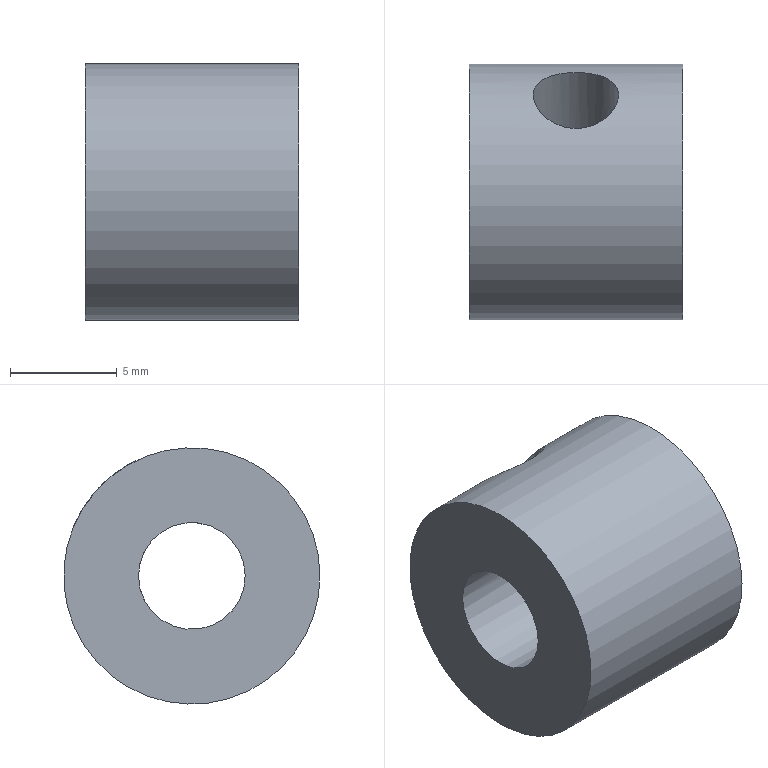Component | NX | 02C__27_2 | 1 solid | 5 faces | volume 889 mm3 | cylinder 3 | plane 2 | commonest cylinder face diameters 12 x1 5 x1 4 x1